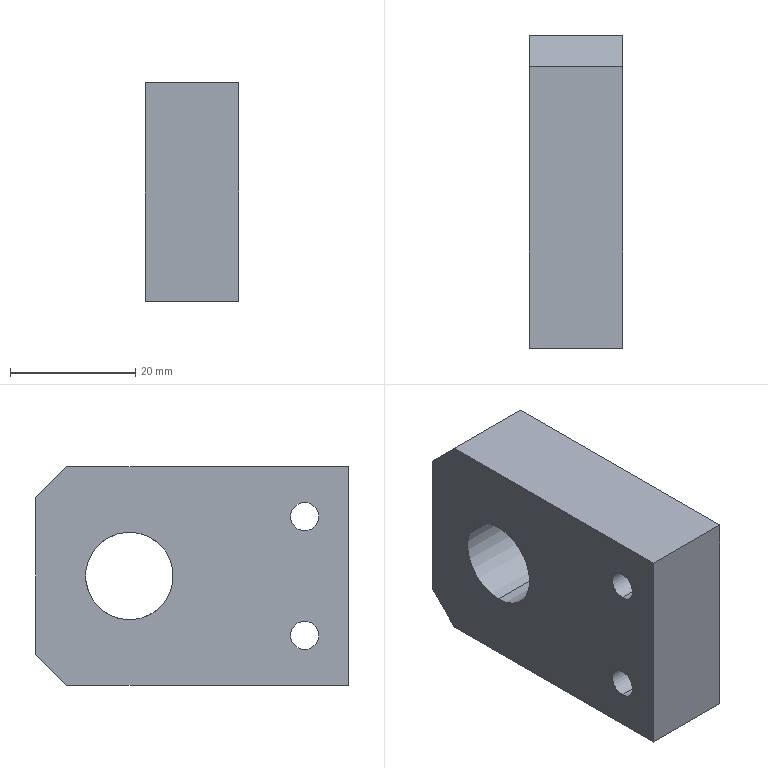Component | SolidWorks | BufferFixingBlock-1 | 1 solid | 20 faces | box 15 x 50 x 35 mm | volume 22786 mm3 | cylinder 10 | plane 10 | commonest cylinder face diameters 8 x4 4.5 x4 14 x2
build123d program:
from build123d import *

# Parameters (mm, degrees)
SKETCH1_2_W                                     = 25
SKETCH1_2_H                                     = 50
BOSS_EXTRUDE1_DEPTH                             = 15
M14X1_5_TAPPED_HOLE1_D                          = 12.5
M14X1_5_TAPPED_HOLE1_DEPTH                      = 32.5
M14X1_5_TAPPED_HOLE1_TIP                        = 3.755
SKETCH6_W                                       = 15
SKETCH6_H                                       = 5
BOSS_EXTRUDE2_DEPTH                             = 50
CHAMFER1_SIZE                                   = 5
M4_HEX_SOCKET_HEAD_CAP_SCREW_CBORE1_D           = 4.5
M4_HEX_SOCKET_HEAD_CAP_SCREW_CBORE1_CBORE_D     = 8
M4_HEX_SOCKET_HEAD_CAP_SCREW_CBORE1_CBORE_DEPTH = 4.4
TAPPEDHOLEMAJORDIA_M14_DEPTH                    = 35.004
TAPPEDHOLEMAJORDIA_M14_DEPTH_BACK               = 35.004
SKETCH1_R                                       = 7


with BuildPart() as part:
    # Sketch1_2 → Boss-Extrude1 (new body)
    with BuildSketch(Plane(origin=(0, 0, 0), x_dir=(0, 0, -1), z_dir=(1, 0, 0))):
        Rectangle(SKETCH1_2_W, SKETCH1_2_H)
    extrude(amount=BOSS_EXTRUDE1_DEPTH)

    # M14x1.5 Tapped Hole1
    with Locations(Plane.ZY):
        with Locations((0, 10)):
            Hole(M14X1_5_TAPPED_HOLE1_D / 2, depth=M14X1_5_TAPPED_HOLE1_DEPTH)
            with Locations((0, 0, -(M14X1_5_TAPPED_HOLE1_DEPTH + M14X1_5_TAPPED_HOLE1_TIP / 2))):  # 118° drill point
                Cone(0, M14X1_5_TAPPED_HOLE1_D / 2, M14X1_5_TAPPED_HOLE1_TIP, mode=Mode.SUBTRACT)

    # Sketch6 → Boss-Extrude2 (add)
    with BuildSketch(Plane.XZ.offset(25)):
        with Locations((7.5, 15)):
            Rectangle(SKETCH6_W, SKETCH6_H)
        with Locations((7.5, -15)):
            Rectangle(SKETCH6_W, SKETCH6_H)
    extrude(amount=-BOSS_EXTRUDE2_DEPTH)

    # Chamfer1
    chamfer1_edges = [part.edges().sort_by_distance(p)[0] for p in [
        (7.5, 25, 17.5),
        (7.5, 25, -17.5),
    ]]
    chamfer(chamfer1_edges, length=CHAMFER1_SIZE)

    # M4 Hex Socket Head Cap Screw CBORE1 (through all)
    with Locations(Plane.ZY):
        with Locations((-9.5, -18), (9.5, -18)):
            CounterBoreHole(M4_HEX_SOCKET_HEAD_CAP_SCREW_CBORE1_D / 2, M4_HEX_SOCKET_HEAD_CAP_SCREW_CBORE1_CBORE_D / 2, M4_HEX_SOCKET_HEAD_CAP_SCREW_CBORE1_CBORE_DEPTH)

    # Sketch1 → TappedHoleMajorDia_M14 (cut, two sides: drawn at the far end of the back side and taken through both)
    with BuildSketch(Plane(origin=(0, 0, 0), x_dir=(0, 0, -1), z_dir=(1, 0, 0)).offset(-TAPPEDHOLEMAJORDIA_M14_DEPTH_BACK)):
        with Locations((0, 10)):
            Circle(SKETCH1_R)
    extrude(amount=TAPPEDHOLEMAJORDIA_M14_DEPTH + TAPPEDHOLEMAJORDIA_M14_DEPTH_BACK, mode=Mode.SUBTRACT)


solid = part.part

# Placed as in the assembly
solid = solid.moved(Location((85, -28.6, -55), (-180, 0, 180)))
STEP:
#1=COLOUR_RGB('',0.7922,0.8196,0.9333);
#2=FILL_AREA_STYLE_COLOUR('',#1);
#3=FILL_AREA_STYLE('',(#2));
#4=SURFACE_STYLE_FILL_AREA(#3);
#5=SURFACE_SIDE_STYLE('',(#4));
#6=SURFACE_STYLE_USAGE(.BOTH.,#5);
#7=PRESENTATION_STYLE_ASSIGNMENT((#6));
#8=CARTESIAN_POINT('',(3.346,-0.7323,-2.441));
#9=VERTEX_POINT('',#8);
#10=CARTESIAN_POINT('',(3.346,-0.7323,-1.89));
#11=VERTEX_POINT('',#10);
#12=CARTESIAN_POINT('',(3.346,-0.7323,-2.441));
#13=CARTESIAN_POINT('',(3.346,-0.7688,-2.441));
#14=CARTESIAN_POINT('',(3.346,-0.804,-2.434));
#15=CARTESIAN_POINT('',(3.346,-0.8715,-2.406));
#16=CARTESIAN_POINT('',(3.346,-0.9013,-2.386));
#17=CARTESIAN_POINT('',(3.346,-0.953,-2.334));
#18=CARTESIAN_POINT('',(3.346,-0.9729,-2.305));
#19=CARTESIAN_POINT('',(3.346,-1.001,-2.237));
#20=CARTESIAN_POINT('',(3.346,-1.008,-2.202));
#21=CARTESIAN_POINT('',(3.346,-1.008,-2.129));
#22=CARTESIAN_POINT('',(3.346,-1.001,-2.094));
#23=CARTESIAN_POINT('',(3.346,-0.9729,-2.026));
#24=CARTESIAN_POINT('',(3.346,-0.953,-1.996));
#25=CARTESIAN_POINT('',(3.346,-0.9013,-1.945));
#26=CARTESIAN_POINT('',(3.346,-0.8715,-1.925));
#27=CARTESIAN_POINT('',(3.346,-0.804,-1.897));
#28=CARTESIAN_POINT('',(3.346,-0.7688,-1.89));
#29=CARTESIAN_POINT('',(3.346,-0.7323,-1.89));
#30=B_SPLINE_CURVE_WITH_KNOTS('',3,(#12,#13,#14,#15,#16,#17,#18,#19,#20,#21,#22,#23,#24,#25,#26,#27,#28,#29),.UNSPECIFIED.,.F.,.F.,(4,2,2,2,2,2,2,2,4),(0.5,0.5625,0.625,0.6875,0.75,0.8125,0.875,0.9375,1.),.UNSPECIFIED.);
#31=EDGE_CURVE('',#9,#11,#30,.T.);
#32=ORIENTED_EDGE('',*,*,#31,.F.);
#33=CARTESIAN_POINT('',(2.756,-0.7323,-2.441));
#34=VERTEX_POINT('',#33);
#35=CARTESIAN_POINT('',(3.346,-0.7323,-2.441));
#36=DIRECTION('',(-1.,0.,0.));
#37=VECTOR('',#36,39.37);
#38=LINE('',#35,#37);
#39=EDGE_CURVE('',#9,#34,#38,.T.);
#40=ORIENTED_EDGE('',*,*,#39,.T.);
#41=CARTESIAN_POINT('',(2.756,-0.7323,-1.89));
#42=VERTEX_POINT('',#41);
#43=CARTESIAN_POINT('',(2.756,-0.7323,-2.165));
#44=DIRECTION('',(-1.,0.,0.));
#45=DIRECTION('',(0.,0.,1.));
#46=AXIS2_PLACEMENT_3D('',#43,#44,#45);
#47=CIRCLE('',#46,0.2756);
#48=EDGE_CURVE('',#34,#42,#47,.T.);
#49=ORIENTED_EDGE('',*,*,#48,.T.);
#50=CARTESIAN_POINT('',(3.346,-0.7323,-1.89));
#51=DIRECTION('',(-1.,0.,0.));
#52=VECTOR('',#51,39.37);
#53=LINE('',#50,#52);
#54=EDGE_CURVE('',#11,#42,#53,.T.);
#55=ORIENTED_EDGE('',*,*,#54,.F.);
#56=EDGE_LOOP('',(#32,#40,#49,#55));
#57=FACE_OUTER_BOUND('',#56,.T.);
#58=CARTESIAN_POINT('',(3.346,-0.7323,-2.165));
#59=DIRECTION('',(-1.,0.,0.));
#60=DIRECTION('',(0.,0.,1.));
#61=AXIS2_PLACEMENT_3D('',#58,#59,#60);
#62=CYLINDRICAL_SURFACE('',#61,0.2756);
#63=ADVANCED_FACE('',(#57),#62,.F.);
#64=CARTESIAN_POINT('',(3.173,-1.835,-1.634));
#65=VERTEX_POINT('',#64);
#66=CARTESIAN_POINT('',(3.173,-1.835,-1.949));
#67=VERTEX_POINT('',#66);
#68=CARTESIAN_POINT('',(3.173,-1.835,-1.791));
#69=DIRECTION('',(1.,-0.,-0.));
#70=DIRECTION('',(0.,0.,-1.));
#71=AXIS2_PLACEMENT_3D('',#68,#69,#70);
#72=CIRCLE('',#71,0.1575);
#73=EDGE_CURVE('',#65,#67,#72,.T.);
#74=ORIENTED_EDGE('',*,*,#73,.F.);
#75=CARTESIAN_POINT('',(3.346,-1.835,-1.634));
#76=VERTEX_POINT('',#75);
#77=CARTESIAN_POINT('',(3.346,-1.835,-1.634));
#78=DIRECTION('',(1.,-0.,-0.));
#79=VECTOR('',#78,39.37);
#80=LINE('',#77,#79);
#81=EDGE_CURVE('',#65,#76,#80,.T.);
#82=ORIENTED_EDGE('',*,*,#81,.T.);
#83=CARTESIAN_POINT('',(3.346,-1.835,-1.949));
#84=VERTEX_POINT('',#83);
#85=CARTESIAN_POINT('',(3.346,-1.835,-1.791));
#86=DIRECTION('',(1.,-0.,-0.));
#87=DIRECTION('',(0.,0.,-1.));
#88=AXIS2_PLACEMENT_3D('',#85,#86,#87);
#89=CIRCLE('',#88,0.1575);
#90=EDGE_CURVE('',#76,#84,#89,.T.);
#91=ORIENTED_EDGE('',*,*,#90,.T.);
#92=CARTESIAN_POINT('',(3.346,-1.835,-1.949));
#93=DIRECTION('',(1.,-0.,-0.));
#94=VECTOR('',#93,39.37);
#95=LINE('',#92,#94);
#96=EDGE_CURVE('',#67,#84,#95,.T.);
#97=ORIENTED_EDGE('',*,*,#96,.F.);
#98=EDGE_LOOP('',(#74,#82,#91,#97));
#99=FACE_OUTER_BOUND('',#98,.T.);
#100=CARTESIAN_POINT('',(3.346,-1.835,-1.791));
#101=DIRECTION('',(1.,-0.,-0.));
#102=DIRECTION('',(0.,0.,-1.));
#103=AXIS2_PLACEMENT_3D('',#100,#101,#102);
#104=CYLINDRICAL_SURFACE('',#103,0.1575);
#105=ADVANCED_FACE('',(#99),#104,.F.);
#106=CARTESIAN_POINT('',(2.756,-1.835,-1.703));
#107=VERTEX_POINT('',#106);
#108=CARTESIAN_POINT('',(2.756,-1.835,-1.88));
#109=VERTEX_POINT('',#108);
#110=CARTESIAN_POINT('',(2.756,-1.835,-1.791));
#111=DIRECTION('',(1.,-0.,-0.));
#112=DIRECTION('',(0.,0.,-1.));
#113=AXIS2_PLACEMENT_3D('',#110,#111,#112);
#114=CIRCLE('',#113,0.08858);
#115=EDGE_CURVE('',#107,#109,#114,.T.);
#116=ORIENTED_EDGE('',*,*,#115,.F.);
#117=CARTESIAN_POINT('',(3.173,-1.835,-1.703));
#118=VERTEX_POINT('',#117);
#119=CARTESIAN_POINT('',(3.346,-1.835,-1.703));
#120=DIRECTION('',(1.,-0.,-0.));
#121=VECTOR('',#120,39.37);
#122=LINE('',#119,#121);
#123=EDGE_CURVE('',#107,#118,#122,.T.);
#124=ORIENTED_EDGE('',*,*,#123,.T.);
#125=CARTESIAN_POINT('',(3.173,-1.835,-1.88));
#126=VERTEX_POINT('',#125);
#127=CARTESIAN_POINT('',(3.173,-1.835,-1.791));
#128=DIRECTION('',(1.,-0.,-0.));
#129=DIRECTION('',(0.,0.,-1.));
#130=AXIS2_PLACEMENT_3D('',#127,#128,#129);
#131=CIRCLE('',#130,0.08858);
#132=EDGE_CURVE('',#118,#126,#131,.T.);
#133=ORIENTED_EDGE('',*,*,#132,.T.);
#134=CARTESIAN_POINT('',(3.346,-1.835,-1.88));
#135=DIRECTION('',(1.,-0.,-0.));
#136=VECTOR('',#135,39.37);
#137=LINE('',#134,#136);
#138=EDGE_CURVE('',#109,#126,#137,.T.);
#139=ORIENTED_EDGE('',*,*,#138,.F.);
#140=EDGE_LOOP('',(#116,#124,#133,#139));
#141=FACE_OUTER_BOUND('',#140,.T.);
#142=CARTESIAN_POINT('',(3.346,-1.835,-1.791));
#143=DIRECTION('',(1.,-0.,-0.));
#144=DIRECTION('',(0.,0.,-1.));
#145=AXIS2_PLACEMENT_3D('',#142,#143,#144);
#146=CYLINDRICAL_SURFACE('',#145,0.08858);
#147=ADVANCED_FACE('',(#141),#146,.F.);
#148=CARTESIAN_POINT('',(3.173,-1.835,-2.382));
#149=VERTEX_POINT('',#148);
#150=CARTESIAN_POINT('',(3.173,-1.835,-2.697));
#151=VERTEX_POINT('',#150);
#152=CARTESIAN_POINT('',(3.173,-1.835,-2.539));
#153=DIRECTION('',(1.,-0.,-0.));
#154=DIRECTION('',(0.,0.,-1.));
#155=AXIS2_PLACEMENT_3D('',#152,#153,#154);
#156=CIRCLE('',#155,0.1575);
#157=EDGE_CURVE('',#149,#151,#156,.T.);
#158=ORIENTED_EDGE('',*,*,#157,.F.);
#159=CARTESIAN_POINT('',(3.346,-1.835,-2.382));
#160=VERTEX_POINT('',#159);
#161=CARTESIAN_POINT('',(3.346,-1.835,-2.382));
#162=DIRECTION('',(1.,-0.,-0.));
#163=VECTOR('',#162,39.37);
#164=LINE('',#161,#163);
#165=EDGE_CURVE('',#149,#160,#164,.T.);
#166=ORIENTED_EDGE('',*,*,#165,.T.);
#167=CARTESIAN_POINT('',(3.346,-1.835,-2.697));
#168=VERTEX_POINT('',#167);
#169=CARTESIAN_POINT('',(3.346,-1.835,-2.539));
#170=DIRECTION('',(1.,-0.,-0.));
#171=DIRECTION('',(0.,0.,-1.));
#172=AXIS2_PLACEMENT_3D('',#169,#170,#171);
#173=CIRCLE('',#172,0.1575);
#174=EDGE_CURVE('',#160,#168,#173,.T.);
#175=ORIENTED_EDGE('',*,*,#174,.T.);
#176=CARTESIAN_POINT('',(3.346,-1.835,-2.697));
#177=DIRECTION('',(1.,-0.,-0.));
#178=VECTOR('',#177,39.37);
#179=LINE('',#176,#178);
#180=EDGE_CURVE('',#151,#168,#179,.T.);
#181=ORIENTED_EDGE('',*,*,#180,.F.);
#182=EDGE_LOOP('',(#158,#166,#175,#181));
#183=FACE_OUTER_BOUND('',#182,.T.);
#184=CARTESIAN_POINT('',(3.346,-1.835,-2.539));
#185=DIRECTION('',(1.,-0.,-0.));
#186=DIRECTION('',(0.,0.,-1.));
#187=AXIS2_PLACEMENT_3D('',#184,#185,#186);
#188=CYLINDRICAL_SURFACE('',#187,0.1575);
#189=ADVANCED_FACE('',(#183),#188,.F.);
#190=CARTESIAN_POINT('',(2.756,-1.835,-2.451));
#191=VERTEX_POINT('',#190);
#192=CARTESIAN_POINT('',(2.756,-1.835,-2.628));
#193=VERTEX_POINT('',#192);
#194=CARTESIAN_POINT('',(2.756,-1.835,-2.539));
#195=DIRECTION('',(1.,-0.,-0.));
#196=DIRECTION('',(0.,0.,-1.));
#197=AXIS2_PLACEMENT_3D('',#194,#195,#196);
#198=CIRCLE('',#197,0.08858);
#199=EDGE_CURVE('',#191,#193,#198,.T.);
#200=ORIENTED_EDGE('',*,*,#199,.F.);
#201=CARTESIAN_POINT('',(3.173,-1.835,-2.451));
#202=VERTEX_POINT('',#201);
#203=CARTESIAN_POINT('',(3.346,-1.835,-2.451));
#204=DIRECTION('',(1.,-0.,-0.));
#205=VECTOR('',#204,39.37);
#206=LINE('',#203,#205);
#207=EDGE_CURVE('',#191,#202,#206,.T.);
#208=ORIENTED_EDGE('',*,*,#207,.T.);
#209=CARTESIAN_POINT('',(3.173,-1.835,-2.628));
#210=VERTEX_POINT('',#209);
#211=CARTESIAN_POINT('',(3.173,-1.835,-2.539));
#212=DIRECTION('',(1.,-0.,-0.));
#213=DIRECTION('',(0.,0.,-1.));
#214=AXIS2_PLACEMENT_3D('',#211,#212,#213);
#215=CIRCLE('',#214,0.08858);
#216=EDGE_CURVE('',#202,#210,#215,.T.);
#217=ORIENTED_EDGE('',*,*,#216,.T.);
#218=CARTESIAN_POINT('',(3.346,-1.835,-2.628));
#219=DIRECTION('',(1.,-0.,-0.));
#220=VECTOR('',#219,39.37);
#221=LINE('',#218,#220);
#222=EDGE_CURVE('',#193,#210,#221,.T.);
#223=ORIENTED_EDGE('',*,*,#222,.F.);
#224=EDGE_LOOP('',(#200,#208,#217,#223));
#225=FACE_OUTER_BOUND('',#224,.T.);
#226=CARTESIAN_POINT('',(3.346,-1.835,-2.539));
#227=DIRECTION('',(1.,-0.,-0.));
#228=DIRECTION('',(0.,0.,-1.));
#229=AXIS2_PLACEMENT_3D('',#226,#227,#228);
#230=CYLINDRICAL_SURFACE('',#229,0.08858);
#231=ADVANCED_FACE('',(#225),#230,.F.);
#232=CARTESIAN_POINT('',(3.346,-2.11,-2.854));
#233=VERTEX_POINT('',#232);
#234=CARTESIAN_POINT('',(3.346,-2.11,-1.476));
#235=VERTEX_POINT('',#234);
#236=CARTESIAN_POINT('',(3.346,-2.11,-1.673));
#237=DIRECTION('',(0.,0.,1.));
#238=VECTOR('',#237,39.37);
#239=LINE('',#236,#238);
#240=EDGE_CURVE('',#233,#235,#239,.T.);
#241=ORIENTED_EDGE('',*,*,#240,.T.);
#242=CARTESIAN_POINT('',(2.756,-2.11,-1.476));
#243=VERTEX_POINT('',#242);
#244=CARTESIAN_POINT('',(3.346,-2.11,-1.476));
#245=DIRECTION('',(-1.,0.,0.));
#246=VECTOR('',#245,39.37);
#247=LINE('',#244,#246);
#248=EDGE_CURVE('',#235,#243,#247,.T.);
#249=ORIENTED_EDGE('',*,*,#248,.T.);
#250=CARTESIAN_POINT('',(2.756,-2.11,-2.854));
#251=VERTEX_POINT('',#250);
#252=CARTESIAN_POINT('',(2.756,-2.11,-1.673));
#253=DIRECTION('',(0.,0.,1.));
#254=VECTOR('',#253,39.37);
#255=LINE('',#252,#254);
#256=EDGE_CURVE('',#251,#243,#255,.T.);
#257=ORIENTED_EDGE('',*,*,#256,.F.);
#258=CARTESIAN_POINT('',(3.346,-2.11,-2.854));
#259=DIRECTION('',(1.,-0.,-0.));
#260=VECTOR('',#259,39.37);
#261=LINE('',#258,#260);
#262=EDGE_CURVE('',#251,#233,#261,.T.);
#263=ORIENTED_EDGE('',*,*,#262,.T.);
#264=EDGE_LOOP('',(#241,#249,#257,#263));
#265=FACE_OUTER_BOUND('',#264,.T.);
#266=CARTESIAN_POINT('',(2.756,-2.11,-1.673));
#267=DIRECTION('',(0.,1.,-0.));
#268=DIRECTION('',(-0.,-0.,-1.));
#269=AXIS2_PLACEMENT_3D('',#266,#267,#268);
#270=PLANE('',#269);
#271=ADVANCED_FACE('',(#265),#270,.F.);
#272=CARTESIAN_POINT('',(2.756,-0.1417,-1.673));
#273=VERTEX_POINT('',#272);
#274=CARTESIAN_POINT('',(2.756,-0.1417,-2.657));
#275=VERTEX_POINT('',#274);
#276=CARTESIAN_POINT('',(2.756,-0.1417,-1.673));
#277=DIRECTION('',(-0.,-0.,-1.));
#278=VECTOR('',#277,39.37);
#279=LINE('',#276,#278);
#280=EDGE_CURVE('',#273,#275,#279,.T.);
#281=ORIENTED_EDGE('',*,*,#280,.F.);
#282=CARTESIAN_POINT('',(3.346,-0.1417,-1.673));
#283=VERTEX_POINT('',#282);
#284=CARTESIAN_POINT('',(3.346,-0.1417,-1.673));
#285=DIRECTION('',(1.,-0.,-0.));
#286=VECTOR('',#285,39.37);
#287=LINE('',#284,#286);
#288=EDGE_CURVE('',#273,#283,#287,.T.);
#289=ORIENTED_EDGE('',*,*,#288,.T.);
#290=CARTESIAN_POINT('',(3.346,-0.1417,-2.657));
#291=VERTEX_POINT('',#290);
#292=CARTESIAN_POINT('',(3.346,-0.1417,-1.673));
#293=DIRECTION('',(-0.,-0.,-1.));
#294=VECTOR('',#293,39.37);
#295=LINE('',#292,#294);
#296=EDGE_CURVE('',#283,#291,#295,.T.);
#297=ORIENTED_EDGE('',*,*,#296,.T.);
#298=CARTESIAN_POINT('',(2.756,-0.1417,-2.657));
#299=DIRECTION('',(-1.,0.,0.));
#300=VECTOR('',#299,39.37);
#301=LINE('',#298,#300);
#302=EDGE_CURVE('',#291,#275,#301,.T.);
#303=ORIENTED_EDGE('',*,*,#302,.T.);
#304=EDGE_LOOP('',(#281,#289,#297,#303));
#305=FACE_OUTER_BOUND('',#304,.T.);
#306=CARTESIAN_POINT('',(2.756,-0.1417,-1.673));
#307=DIRECTION('',(-0.,-1.,0.));
#308=DIRECTION('',(0.,0.,1.));
#309=AXIS2_PLACEMENT_3D('',#306,#307,#308);
#310=PLANE('',#309);
#311=ADVANCED_FACE('',(#305),#310,.F.);
#312=CARTESIAN_POINT('',(2.756,-0.7323,-2.165));
#313=DIRECTION('',(-1.,0.,0.));
#314=DIRECTION('',(0.,0.,1.));
#315=AXIS2_PLACEMENT_3D('',#312,#313,#314);
#316=CIRCLE('',#315,0.2756);
#317=EDGE_CURVE('',#42,#34,#316,.T.);
#318=ORIENTED_EDGE('',*,*,#317,.F.);
#319=ORIENTED_EDGE('',*,*,#48,.F.);
#320=EDGE_LOOP('',(#318,#319));
#321=FACE_BOUND('',#320,.T.);
#322=CARTESIAN_POINT('',(2.756,-1.835,-1.791));
#323=DIRECTION('',(1.,-0.,-0.));
#324=DIRECTION('',(0.,0.,-1.));
#325=AXIS2_PLACEMENT_3D('',#322,#323,#324);
#326=CIRCLE('',#325,0.08858);
#327=EDGE_CURVE('',#109,#107,#326,.T.);
#328=ORIENTED_EDGE('',*,*,#327,.T.);
#329=ORIENTED_EDGE('',*,*,#115,.T.);
#330=EDGE_LOOP('',(#328,#329));
#331=FACE_BOUND('',#330,.T.);
#332=CARTESIAN_POINT('',(2.756,-1.835,-2.539));
#333=DIRECTION('',(1.,-0.,-0.));
#334=DIRECTION('',(0.,0.,-1.));
#335=AXIS2_PLACEMENT_3D('',#332,#333,#334);
#336=CIRCLE('',#335,0.08858);
#337=EDGE_CURVE('',#193,#191,#336,.T.);
#338=ORIENTED_EDGE('',*,*,#337,.T.);
#339=ORIENTED_EDGE('',*,*,#199,.T.);
#340=EDGE_LOOP('',(#338,#339));
#341=FACE_BOUND('',#340,.T.);
#342=CARTESIAN_POINT('',(2.756,-0.3386,-1.476));
#343=VERTEX_POINT('',#342);
#344=CARTESIAN_POINT('',(2.756,-0.1417,-1.476));
#345=DIRECTION('',(-0.,-1.,0.));
#346=VECTOR('',#345,39.37);
#347=LINE('',#344,#346);
#348=EDGE_CURVE('',#343,#243,#347,.T.);
#349=ORIENTED_EDGE('',*,*,#348,.F.);
#350=CARTESIAN_POINT('',(2.756,-0.3878,-1.427));
#351=DIRECTION('',(-0.,0.7071,-0.7071));
#352=VECTOR('',#351,39.37);
#353=LINE('',#350,#352);
#354=EDGE_CURVE('',#343,#273,#353,.T.);
#355=ORIENTED_EDGE('',*,*,#354,.T.);
#356=ORIENTED_EDGE('',*,*,#280,.T.);
#357=CARTESIAN_POINT('',(2.756,-0.3386,-2.854));
#358=VERTEX_POINT('',#357);
#359=CARTESIAN_POINT('',(2.756,-0.3878,-2.904));
#360=DIRECTION('',(-0.,-0.7071,-0.7071));
#361=VECTOR('',#360,39.37);
#362=LINE('',#359,#361);
#363=EDGE_CURVE('',#275,#358,#362,.T.);
#364=ORIENTED_EDGE('',*,*,#363,.T.);
#365=CARTESIAN_POINT('',(2.756,-0.1417,-2.854));
#366=DIRECTION('',(-0.,-1.,0.));
#367=VECTOR('',#366,39.37);
#368=LINE('',#365,#367);
#369=EDGE_CURVE('',#358,#251,#368,.T.);
#370=ORIENTED_EDGE('',*,*,#369,.T.);
#371=ORIENTED_EDGE('',*,*,#256,.T.);
#372=EDGE_LOOP('',(#349,#355,#356,#364,#370,#371));
#373=FACE_OUTER_BOUND('',#372,.T.);
#374=CARTESIAN_POINT('',(2.756,-1.126,-2.165));
#375=DIRECTION('',(-1.,0.,0.));
#376=DIRECTION('',(0.,0.,1.));
#377=AXIS2_PLACEMENT_3D('',#374,#375,#376);
#378=PLANE('',#377);
#379=ADVANCED_FACE('',(#321,#331,#341,#373),#378,.T.);
#380=CARTESIAN_POINT('',(3.346,-0.7323,-1.89));
#381=CARTESIAN_POINT('',(3.346,-0.6957,-1.89));
#382=CARTESIAN_POINT('',(3.346,-0.6606,-1.897));
#383=CARTESIAN_POINT('',(3.346,-0.5931,-1.925));
#384=CARTESIAN_POINT('',(3.346,-0.5632,-1.945));
#385=CARTESIAN_POINT('',(3.346,-0.5116,-1.996));
#386=CARTESIAN_POINT('',(3.346,-0.4917,-2.026));
#387=CARTESIAN_POINT('',(3.346,-0.4637,-2.094));
#388=CARTESIAN_POINT('',(3.346,-0.4567,-2.129));
#389=CARTESIAN_POINT('',(3.346,-0.4567,-2.202));
#390=CARTESIAN_POINT('',(3.346,-0.4637,-2.237));
#391=CARTESIAN_POINT('',(3.346,-0.4916,-2.305));
#392=CARTESIAN_POINT('',(3.346,-0.5116,-2.334));
#393=CARTESIAN_POINT('',(3.346,-0.5632,-2.386));
#394=CARTESIAN_POINT('',(3.346,-0.5931,-2.406));
#395=CARTESIAN_POINT('',(3.346,-0.6606,-2.434));
#396=CARTESIAN_POINT('',(3.346,-0.6958,-2.441));
#397=CARTESIAN_POINT('',(3.346,-0.7323,-2.441));
#398=B_SPLINE_CURVE_WITH_KNOTS('',3,(#380,#381,#382,#383,#384,#385,#386,#387,#388,#389,#390,#391,#392,#393,#394,#395,#396,#397),.UNSPECIFIED.,.F.,.F.,(4,2,2,2,2,2,2,2,4),(0.,0.0625,0.125,0.1875,0.25,0.3125,0.375,0.4375,0.5),.UNSPECIFIED.);
#399=EDGE_CURVE('',#11,#9,#398,.T.);
#400=ORIENTED_EDGE('',*,*,#399,.T.);
#401=ORIENTED_EDGE('',*,*,#31,.T.);
#402=EDGE_LOOP('',(#400,#401));
#403=FACE_BOUND('',#402,.T.);
#404=CARTESIAN_POINT('',(3.346,-1.835,-1.791));
#405=DIRECTION('',(1.,-0.,-0.));
#406=DIRECTION('',(0.,0.,-1.));
#407=AXIS2_PLACEMENT_3D('',#404,#405,#406);
#408=CIRCLE('',#407,0.1575);
#409=EDGE_CURVE('',#84,#76,#408,.T.);
#410=ORIENTED_EDGE('',*,*,#409,.F.);
#411=ORIENTED_EDGE('',*,*,#90,.F.);
#412=EDGE_LOOP('',(#410,#411));
#413=FACE_BOUND('',#412,.T.);
#414=CARTESIAN_POINT('',(3.346,-1.835,-2.539));
#415=DIRECTION('',(1.,-0.,-0.));
#416=DIRECTION('',(0.,0.,-1.));
#417=AXIS2_PLACEMENT_3D('',#414,#415,#416);
#418=CIRCLE('',#417,0.1575);
#419=EDGE_CURVE('',#168,#160,#418,.T.);
#420=ORIENTED_EDGE('',*,*,#419,.F.);
#421=ORIENTED_EDGE('',*,*,#174,.F.);
#422=EDGE_LOOP('',(#420,#421));
#423=FACE_BOUND('',#422,.T.);
#424=ORIENTED_EDGE('',*,*,#296,.F.);
#425=CARTESIAN_POINT('',(3.346,-0.3386,-1.476));
#426=VERTEX_POINT('',#425);
#427=CARTESIAN_POINT('',(3.346,-0.3386,-1.476));
#428=DIRECTION('',(0.,-0.7071,0.7071));
#429=VECTOR('',#428,39.37);
#430=LINE('',#427,#429);
#431=EDGE_CURVE('',#283,#426,#430,.T.);
#432=ORIENTED_EDGE('',*,*,#431,.T.);
#433=CARTESIAN_POINT('',(3.346,-0.1417,-1.476));
#434=DIRECTION('',(-0.,-1.,0.));
#435=VECTOR('',#434,39.37);
#436=LINE('',#433,#435);
#437=EDGE_CURVE('',#426,#235,#436,.T.);
#438=ORIENTED_EDGE('',*,*,#437,.T.);
#439=ORIENTED_EDGE('',*,*,#240,.F.);
#440=CARTESIAN_POINT('',(3.346,-0.3386,-2.854));
#441=VERTEX_POINT('',#440);
#442=CARTESIAN_POINT('',(3.346,-0.1417,-2.854));
#443=DIRECTION('',(-0.,-1.,0.));
#444=VECTOR('',#443,39.37);
#445=LINE('',#442,#444);
#446=EDGE_CURVE('',#441,#233,#445,.T.);
#447=ORIENTED_EDGE('',*,*,#446,.F.);
#448=CARTESIAN_POINT('',(3.346,-0.3386,-2.854));
#449=DIRECTION('',(0.,0.7071,0.7071));
#450=VECTOR('',#449,39.37);
#451=LINE('',#448,#450);
#452=EDGE_CURVE('',#441,#291,#451,.T.);
#453=ORIENTED_EDGE('',*,*,#452,.T.);
#454=EDGE_LOOP('',(#424,#432,#438,#439,#447,#453));
#455=FACE_OUTER_BOUND('',#454,.T.);
#456=CARTESIAN_POINT('',(3.346,-1.126,-2.165));
#457=DIRECTION('',(-1.,0.,0.));
#458=DIRECTION('',(0.,0.,1.));
#459=AXIS2_PLACEMENT_3D('',#456,#457,#458);
#460=PLANE('',#459);
#461=ADVANCED_FACE('',(#403,#413,#423,#455),#460,.F.);
#462=ORIENTED_EDGE('',*,*,#369,.F.);
#463=CARTESIAN_POINT('',(3.346,-0.3386,-2.854));
#464=DIRECTION('',(1.,-0.,-0.));
#465=VECTOR('',#464,39.37);
#466=LINE('',#463,#465);
#467=EDGE_CURVE('',#358,#441,#466,.T.);
#468=ORIENTED_EDGE('',*,*,#467,.T.);
#469=ORIENTED_EDGE('',*,*,#446,.T.);
#470=ORIENTED_EDGE('',*,*,#262,.F.);
#471=EDGE_LOOP('',(#462,#468,#469,#470));
#472=FACE_OUTER_BOUND('',#471,.T.);
#473=CARTESIAN_POINT('',(3.346,-0.1417,-2.854));
#474=DIRECTION('',(-0.,-0.,-1.));
#475=DIRECTION('',(-0.,-1.,0.));
#476=AXIS2_PLACEMENT_3D('',#473,#474,#475);
#477=PLANE('',#476);
#478=ADVANCED_FACE('',(#472),#477,.T.);
#479=ORIENTED_EDGE('',*,*,#437,.F.);
#480=CARTESIAN_POINT('',(2.756,-0.3386,-1.476));
#481=DIRECTION('',(-1.,0.,0.));
#482=VECTOR('',#481,39.37);
#483=LINE('',#480,#482);
#484=EDGE_CURVE('',#426,#343,#483,.T.);
#485=ORIENTED_EDGE('',*,*,#484,.T.);
#486=ORIENTED_EDGE('',*,*,#348,.T.);
#487=ORIENTED_EDGE('',*,*,#248,.F.);
#488=EDGE_LOOP('',(#479,#485,#486,#487));
#489=FACE_OUTER_BOUND('',#488,.T.);
#490=CARTESIAN_POINT('',(3.346,-0.1417,-1.476));
#491=DIRECTION('',(0.,0.,1.));
#492=DIRECTION('',(0.,1.,-0.));
#493=AXIS2_PLACEMENT_3D('',#490,#491,#492);
#494=PLANE('',#493);
#495=ADVANCED_FACE('',(#489),#494,.T.);
#496=ORIENTED_EDGE('',*,*,#431,.F.);
#497=ORIENTED_EDGE('',*,*,#288,.F.);
#498=ORIENTED_EDGE('',*,*,#354,.F.);
#499=ORIENTED_EDGE('',*,*,#484,.F.);
#500=EDGE_LOOP('',(#496,#497,#498,#499));
#501=FACE_OUTER_BOUND('',#500,.T.);
#502=CARTESIAN_POINT('',(3.346,-0.3386,-1.476));
#503=DIRECTION('',(0.,0.7071,0.7071));
#504=DIRECTION('',(1.,-0.,-0.));
#505=AXIS2_PLACEMENT_3D('',#502,#503,#504);
#506=PLANE('',#505);
#507=ADVANCED_FACE('',(#501),#506,.T.);
#508=ORIENTED_EDGE('',*,*,#363,.F.);
#509=ORIENTED_EDGE('',*,*,#302,.F.);
#510=ORIENTED_EDGE('',*,*,#452,.F.);
#511=ORIENTED_EDGE('',*,*,#467,.F.);
#512=EDGE_LOOP('',(#508,#509,#510,#511));
#513=FACE_OUTER_BOUND('',#512,.T.);
#514=CARTESIAN_POINT('',(3.346,-0.3386,-2.854));
#515=DIRECTION('',(0.,0.7071,-0.7071));
#516=DIRECTION('',(-1.,0.,0.));
#517=AXIS2_PLACEMENT_3D('',#514,#515,#516);
#518=PLANE('',#517);
#519=ADVANCED_FACE('',(#513),#518,.T.);
#520=ORIENTED_EDGE('',*,*,#207,.F.);
#521=ORIENTED_EDGE('',*,*,#337,.F.);
#522=ORIENTED_EDGE('',*,*,#222,.T.);
#523=CARTESIAN_POINT('',(3.173,-1.835,-2.539));
#524=DIRECTION('',(1.,-0.,-0.));
#525=DIRECTION('',(0.,0.,-1.));
#526=AXIS2_PLACEMENT_3D('',#523,#524,#525);
#527=CIRCLE('',#526,0.08858);
#528=EDGE_CURVE('',#210,#202,#527,.T.);
#529=ORIENTED_EDGE('',*,*,#528,.T.);
#530=EDGE_LOOP('',(#520,#521,#522,#529));
#531=FACE_OUTER_BOUND('',#530,.T.);
#532=CARTESIAN_POINT('',(3.346,-1.835,-2.539));
#533=DIRECTION('',(1.,-0.,-0.));
#534=DIRECTION('',(0.,0.,-1.));
#535=AXIS2_PLACEMENT_3D('',#532,#533,#534);
#536=CYLINDRICAL_SURFACE('',#535,0.08858);
#537=ADVANCED_FACE('',(#531),#536,.F.);
#538=ORIENTED_EDGE('',*,*,#528,.F.);
#539=ORIENTED_EDGE('',*,*,#216,.F.);
#540=EDGE_LOOP('',(#538,#539));
#541=FACE_BOUND('',#540,.T.);
#542=CARTESIAN_POINT('',(3.173,-1.835,-2.539));
#543=DIRECTION('',(1.,-0.,-0.));
#544=DIRECTION('',(0.,0.,-1.));
#545=AXIS2_PLACEMENT_3D('',#542,#543,#544);
#546=CIRCLE('',#545,0.1575);
#547=EDGE_CURVE('',#151,#149,#546,.T.);
#548=ORIENTED_EDGE('',*,*,#547,.T.);
#549=ORIENTED_EDGE('',*,*,#157,.T.);
#550=EDGE_LOOP('',(#548,#549));
#551=FACE_OUTER_BOUND('',#550,.T.);
#552=CARTESIAN_POINT('',(3.173,-1.746,-2.539));
#553=DIRECTION('',(-1.,0.,0.));
#554=DIRECTION('',(0.,0.,1.));
#555=AXIS2_PLACEMENT_3D('',#552,#553,#554);
#556=PLANE('',#555);
#557=ADVANCED_FACE('',(#541,#551),#556,.F.);
#558=ORIENTED_EDGE('',*,*,#165,.F.);
#559=ORIENTED_EDGE('',*,*,#547,.F.);
#560=ORIENTED_EDGE('',*,*,#180,.T.);
#561=ORIENTED_EDGE('',*,*,#419,.T.);
#562=EDGE_LOOP('',(#558,#559,#560,#561));
#563=FACE_OUTER_BOUND('',#562,.T.);
#564=CARTESIAN_POINT('',(3.346,-1.835,-2.539));
#565=DIRECTION('',(1.,-0.,-0.));
#566=DIRECTION('',(0.,0.,-1.));
#567=AXIS2_PLACEMENT_3D('',#564,#565,#566);
#568=CYLINDRICAL_SURFACE('',#567,0.1575);
#569=ADVANCED_FACE('',(#563),#568,.F.);
#570=ORIENTED_EDGE('',*,*,#123,.F.);
#571=ORIENTED_EDGE('',*,*,#327,.F.);
#572=ORIENTED_EDGE('',*,*,#138,.T.);
#573=CARTESIAN_POINT('',(3.173,-1.835,-1.791));
#574=DIRECTION('',(1.,-0.,-0.));
#575=DIRECTION('',(0.,0.,-1.));
#576=AXIS2_PLACEMENT_3D('',#573,#574,#575);
#577=CIRCLE('',#576,0.08858);
#578=EDGE_CURVE('',#126,#118,#577,.T.);
#579=ORIENTED_EDGE('',*,*,#578,.T.);
#580=EDGE_LOOP('',(#570,#571,#572,#579));
#581=FACE_OUTER_BOUND('',#580,.T.);
#582=CARTESIAN_POINT('',(3.346,-1.835,-1.791));
#583=DIRECTION('',(1.,-0.,-0.));
#584=DIRECTION('',(0.,0.,-1.));
#585=AXIS2_PLACEMENT_3D('',#582,#583,#584);
#586=CYLINDRICAL_SURFACE('',#585,0.08858);
#587=ADVANCED_FACE('',(#581),#586,.F.);
#588=ORIENTED_EDGE('',*,*,#578,.F.);
#589=ORIENTED_EDGE('',*,*,#132,.F.);
#590=EDGE_LOOP('',(#588,#589));
#591=FACE_BOUND('',#590,.T.);
#592=CARTESIAN_POINT('',(3.173,-1.835,-1.791));
#593=DIRECTION('',(1.,-0.,-0.));
#594=DIRECTION('',(0.,0.,-1.));
#595=AXIS2_PLACEMENT_3D('',#592,#593,#594);
#596=CIRCLE('',#595,0.1575);
#597=EDGE_CURVE('',#67,#65,#596,.T.);
#598=ORIENTED_EDGE('',*,*,#597,.T.);
#599=ORIENTED_EDGE('',*,*,#73,.T.);
#600=EDGE_LOOP('',(#598,#599));
#601=FACE_OUTER_BOUND('',#600,.T.);
#602=CARTESIAN_POINT('',(3.173,-1.746,-1.791));
#603=DIRECTION('',(-1.,0.,0.));
#604=DIRECTION('',(0.,0.,1.));
#605=AXIS2_PLACEMENT_3D('',#602,#603,#604);
#606=PLANE('',#605);
#607=ADVANCED_FACE('',(#591,#601),#606,.F.);
#608=ORIENTED_EDGE('',*,*,#81,.F.);
#609=ORIENTED_EDGE('',*,*,#597,.F.);
#610=ORIENTED_EDGE('',*,*,#96,.T.);
#611=ORIENTED_EDGE('',*,*,#409,.T.);
#612=EDGE_LOOP('',(#608,#609,#610,#611));
#613=FACE_OUTER_BOUND('',#612,.T.);
#614=CARTESIAN_POINT('',(3.346,-1.835,-1.791));
#615=DIRECTION('',(1.,-0.,-0.));
#616=DIRECTION('',(0.,0.,-1.));
#617=AXIS2_PLACEMENT_3D('',#614,#615,#616);
#618=CYLINDRICAL_SURFACE('',#617,0.1575);
#619=ADVANCED_FACE('',(#613),#618,.F.);
#620=ORIENTED_EDGE('',*,*,#39,.F.);
#621=ORIENTED_EDGE('',*,*,#399,.F.);
#622=ORIENTED_EDGE('',*,*,#54,.T.);
#623=ORIENTED_EDGE('',*,*,#317,.T.);
#624=EDGE_LOOP('',(#620,#621,#622,#623));
#625=FACE_OUTER_BOUND('',#624,.T.);
#626=CARTESIAN_POINT('',(3.346,-0.7323,-2.165));
#627=DIRECTION('',(-1.,0.,0.));
#628=DIRECTION('',(0.,0.,1.));
#629=AXIS2_PLACEMENT_3D('',#626,#627,#628);
#630=CYLINDRICAL_SURFACE('',#629,0.2756);
#631=ADVANCED_FACE('',(#625),#630,.F.);
#632=CLOSED_SHELL('',(#63,#105,#147,#189,#231,#271,#311,#379,#461,#478,#495,#507,#519,#537,#557,#569,#587,#607,#619,#631));
#633=MANIFOLD_SOLID_BREP('',#632);
#634=STYLED_ITEM('',(#7),#633);
#635=PRESENTATION_LAYER_ASSIGNMENT('','',(#634));
#636=(LENGTH_UNIT()NAMED_UNIT(*)SI_UNIT($,.METRE.));
#637=LENGTH_MEASURE_WITH_UNIT(LENGTH_MEASURE(0.0254),#636);
#638=DIMENSIONAL_EXPONENTS(1.,0.,0.,0.,0.,0.,0.);
#639=(CONVERSION_BASED_UNIT('',#637)LENGTH_UNIT()NAMED_UNIT(#638));
#640=UNCERTAINTY_MEASURE_WITH_UNIT(LENGTH_MEASURE(0.00001),#639,'','');
#641=(NAMED_UNIT(*)PLANE_ANGLE_UNIT()SI_UNIT($,.RADIAN.));
#642=(NAMED_UNIT(*)SI_UNIT($,.STERADIAN.)SOLID_ANGLE_UNIT());
#643=(GEOMETRIC_REPRESENTATION_CONTEXT(3)GLOBAL_UNCERTAINTY_ASSIGNED_CONTEXT((#640))GLOBAL_UNIT_ASSIGNED_CONTEXT((#639,#641,#642))REPRESENTATION_CONTEXT('',''));
#644=MECHANICAL_DESIGN_GEOMETRIC_PRESENTATION_REPRESENTATION('',(#634),#643);
#645=CARTESIAN_POINT('',(0.,0.,0.));
#646=DIRECTION('',(0.,0.,1.));
#647=DIRECTION('',(1.,0.,0.));
#648=AXIS2_PLACEMENT_3D('',#645,#646,#647);
#649=(LENGTH_UNIT()NAMED_UNIT(*)SI_UNIT($,.METRE.));
#650=LENGTH_MEASURE_WITH_UNIT(LENGTH_MEASURE(0.0254),#649);
#651=DIMENSIONAL_EXPONENTS(1.,0.,0.,0.,0.,0.,0.);
#652=(CONVERSION_BASED_UNIT('',#650)LENGTH_UNIT()NAMED_UNIT(#651));
#653=UNCERTAINTY_MEASURE_WITH_UNIT(LENGTH_MEASURE(0.00001),#652,'','');
#654=(NAMED_UNIT(*)PLANE_ANGLE_UNIT()SI_UNIT($,.RADIAN.));
#655=(NAMED_UNIT(*)SI_UNIT($,.STERADIAN.)SOLID_ANGLE_UNIT());
#656=(GEOMETRIC_REPRESENTATION_CONTEXT(3)GLOBAL_UNCERTAINTY_ASSIGNED_CONTEXT((#653))GLOBAL_UNIT_ASSIGNED_CONTEXT((#652,#654,#655))REPRESENTATION_CONTEXT('',''));
#657=ADVANCED_BREP_SHAPE_REPRESENTATION('',(#633,#648),#656);